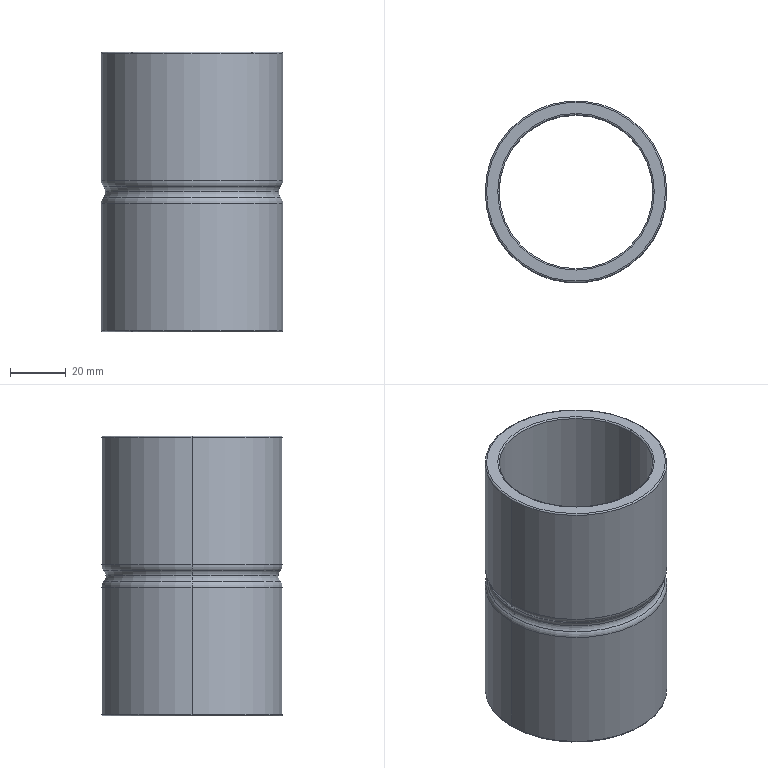Component | SolidWorks | KLHFH007_18LocatingPinSeatBrassSleeve-1 | 1 solid | 24 faces | box 65 x 65 x 100 mm | volume 93014 mm3 | torus 16 | cylinder 6 | plane 2 | commonest cylinder face diameters 65 x4 55 x2 | material Brass
build123d program:
from build123d import *

# Parameters (mm, degrees)
SKETCH1_R           = 32.5
SKETCH1_R_2         = 27.5
BOSS_EXTRUDE1_DEPTH = 50
SKETCH2_R           = 3
FILLET1_R           = 0.5
FILLET2_R           = 3


with BuildPart() as part:
    # Sketch1 → Boss-Extrude1 (new, symmetric)
    with BuildSketch(Plane.XY):
        Circle(SKETCH1_R)
        Circle(SKETCH1_R_2, mode=Mode.SUBTRACT)
    extrude(amount=BOSS_EXTRUDE1_DEPTH, both=True)

    # Sketch2 → Cut-Revolve1 (revolve, cut)
    with BuildSketch(Plane(origin=(0, 0, 0), x_dir=(0, 0, -1), z_dir=(1, 0, 0)), mode=Mode.PRIVATE) as cut_revolve1_sk:
        with Locations((0, 34)):
            Circle(SKETCH2_R)
    revolve(cut_revolve1_sk.sketch.rotate(Axis((0, 0, 0), (0, 0, 1)), 90), axis=Axis((0, 0, 0), (0, 0, 1)), mode=Mode.SUBTRACT)

    # Fillet1
    fillet1_edges = [part.edges().sort_by_distance(p)[0] for p in [
        (-32.5, 0, -50),
        (-32.5, 0, 50),
        (-27.5, 0, -50),
        (-27.5, 0, 50),
    ]]
    fillet(fillet1_edges, radius=FILLET1_R)

    # Fillet2
    fillet2_edges = [part.edges().sort_by_distance(p)[0] for p in [
        (0, 32.5, 2.598),
        (0, 32.5, -2.598),
    ]]
    fillet(fillet2_edges, radius=FILLET2_R)


solid = part.part

# Placed as in the assembly
solid = solid.moved(Location((91, 157.617, -294.5), (0, 0, 0)))
STEP:
#1=CARTESIAN_POINT('',(2.333,6.205,-11.673));
#2=VERTEX_POINT('',#1);
#3=CARTESIAN_POINT('',(2.362,6.205,-11.594));
#4=VERTEX_POINT('',#3);
#5=CARTESIAN_POINT('',(2.244,6.205,-11.594));
#6=DIRECTION('',(0.,-1.,0.));
#7=DIRECTION('',(0.,0.,-1.));
#8=AXIS2_PLACEMENT_3D('',#5,#6,#7);
#9=CIRCLE('',#8,0.1181);
#10=EDGE_CURVE('',#2,#4,#9,.T.);
#11=ORIENTED_EDGE('',*,*,#10,.T.);
#12=CARTESIAN_POINT('',(4.803,6.205,-11.594));
#13=VERTEX_POINT('',#12);
#14=CARTESIAN_POINT('',(3.583,6.205,-11.594));
#15=DIRECTION('',(0.,0.,-1.));
#16=DIRECTION('',(-1.,0.,0.));
#17=AXIS2_PLACEMENT_3D('',#14,#15,#16);
#18=CIRCLE('',#17,1.22);
#19=EDGE_CURVE('',#4,#13,#18,.T.);
#20=ORIENTED_EDGE('',*,*,#19,.T.);
#21=CARTESIAN_POINT('',(4.833,6.205,-11.673));
#22=VERTEX_POINT('',#21);
#23=CARTESIAN_POINT('',(4.921,6.205,-11.594));
#24=DIRECTION('',(-0.,1.,0.));
#25=DIRECTION('',(-1.,0.,0.));
#26=AXIS2_PLACEMENT_3D('',#23,#24,#25);
#27=CIRCLE('',#26,0.1181);
#28=EDGE_CURVE('',#22,#13,#27,.T.);
#29=ORIENTED_EDGE('',*,*,#28,.F.);
#30=CARTESIAN_POINT('',(3.583,6.205,-11.673));
#31=DIRECTION('',(0.,0.,1.));
#32=DIRECTION('',(1.,0.,0.));
#33=AXIS2_PLACEMENT_3D('',#30,#31,#32);
#34=CIRCLE('',#33,1.25);
#35=EDGE_CURVE('',#22,#2,#34,.T.);
#36=ORIENTED_EDGE('',*,*,#35,.T.);
#37=EDGE_LOOP('',(#11,#20,#29,#36));
#38=FACE_OUTER_BOUND('',#37,.T.);
#39=CARTESIAN_POINT('',(3.583,6.205,-11.594));
#40=DIRECTION('',(0.,0.,-1.));
#41=DIRECTION('',(-1.,0.,0.));
#42=AXIS2_PLACEMENT_3D('',#39,#40,#41);
#43=TOROIDAL_SURFACE('',#42,1.339,0.1181);
#44=ADVANCED_FACE('',(#38),#43,.F.);
#45=ORIENTED_EDGE('',*,*,#28,.T.);
#46=CARTESIAN_POINT('',(3.583,6.205,-11.594));
#47=DIRECTION('',(0.,0.,-1.));
#48=DIRECTION('',(-1.,0.,0.));
#49=AXIS2_PLACEMENT_3D('',#46,#47,#48);
#50=CIRCLE('',#49,1.22);
#51=EDGE_CURVE('',#13,#4,#50,.T.);
#52=ORIENTED_EDGE('',*,*,#51,.T.);
#53=ORIENTED_EDGE('',*,*,#10,.F.);
#54=CARTESIAN_POINT('',(3.583,6.205,-11.673));
#55=DIRECTION('',(0.,0.,1.));
#56=DIRECTION('',(1.,0.,0.));
#57=AXIS2_PLACEMENT_3D('',#54,#55,#56);
#58=CIRCLE('',#57,1.25);
#59=EDGE_CURVE('',#2,#22,#58,.T.);
#60=ORIENTED_EDGE('',*,*,#59,.T.);
#61=EDGE_LOOP('',(#45,#52,#53,#60));
#62=FACE_OUTER_BOUND('',#61,.T.);
#63=CARTESIAN_POINT('',(3.583,6.205,-11.594));
#64=DIRECTION('',(0.,0.,-1.));
#65=DIRECTION('',(-1.,0.,0.));
#66=AXIS2_PLACEMENT_3D('',#63,#64,#65);
#67=TOROIDAL_SURFACE('',#66,1.339,0.1181);
#68=ADVANCED_FACE('',(#62),#67,.F.);
#69=CARTESIAN_POINT('',(2.303,6.205,-11.751));
#70=VERTEX_POINT('',#69);
#71=CARTESIAN_POINT('',(4.862,6.205,-11.751));
#72=VERTEX_POINT('',#71);
#73=CARTESIAN_POINT('',(3.583,6.205,-11.751));
#74=DIRECTION('',(0.,0.,-1.));
#75=DIRECTION('',(1.,0.,0.));
#76=AXIS2_PLACEMENT_3D('',#73,#74,#75);
#77=CIRCLE('',#76,1.28);
#78=EDGE_CURVE('',#70,#72,#77,.T.);
#79=ORIENTED_EDGE('',*,*,#78,.F.);
#80=CARTESIAN_POINT('',(2.421,6.205,-11.751));
#81=DIRECTION('',(0.,1.,0.));
#82=DIRECTION('',(-1.,0.,0.));
#83=AXIS2_PLACEMENT_3D('',#80,#81,#82);
#84=CIRCLE('',#83,0.1181);
#85=EDGE_CURVE('',#70,#2,#84,.T.);
#86=ORIENTED_EDGE('',*,*,#85,.T.);
#87=ORIENTED_EDGE('',*,*,#35,.F.);
#88=CARTESIAN_POINT('',(4.744,6.205,-11.751));
#89=DIRECTION('',(0.,-1.,0.));
#90=DIRECTION('',(0.,0.,-1.));
#91=AXIS2_PLACEMENT_3D('',#88,#89,#90);
#92=CIRCLE('',#91,0.1181);
#93=EDGE_CURVE('',#72,#22,#92,.T.);
#94=ORIENTED_EDGE('',*,*,#93,.F.);
#95=EDGE_LOOP('',(#79,#86,#87,#94));
#96=FACE_OUTER_BOUND('',#95,.T.);
#97=CARTESIAN_POINT('',(3.583,6.205,-11.751));
#98=DIRECTION('',(0.,0.,1.));
#99=DIRECTION('',(1.,0.,0.));
#100=AXIS2_PLACEMENT_3D('',#97,#98,#99);
#101=TOROIDAL_SURFACE('',#100,1.161,0.1181);
#102=ADVANCED_FACE('',(#96),#101,.T.);
#103=CARTESIAN_POINT('',(4.862,6.205,-11.438));
#104=VERTEX_POINT('',#103);
#105=CARTESIAN_POINT('',(2.303,6.205,-11.438));
#106=VERTEX_POINT('',#105);
#107=CARTESIAN_POINT('',(3.583,6.205,-11.438));
#108=DIRECTION('',(0.,0.,1.));
#109=DIRECTION('',(-1.,0.,0.));
#110=AXIS2_PLACEMENT_3D('',#107,#108,#109);
#111=CIRCLE('',#110,1.28);
#112=EDGE_CURVE('',#104,#106,#111,.T.);
#113=ORIENTED_EDGE('',*,*,#112,.F.);
#114=CARTESIAN_POINT('',(4.833,6.205,-11.516));
#115=VERTEX_POINT('',#114);
#116=CARTESIAN_POINT('',(4.744,6.205,-11.438));
#117=DIRECTION('',(-0.,1.,0.));
#118=DIRECTION('',(-1.,0.,0.));
#119=AXIS2_PLACEMENT_3D('',#116,#117,#118);
#120=CIRCLE('',#119,0.1181);
#121=EDGE_CURVE('',#104,#115,#120,.T.);
#122=ORIENTED_EDGE('',*,*,#121,.T.);
#123=CARTESIAN_POINT('',(2.333,6.205,-11.516));
#124=VERTEX_POINT('',#123);
#125=CARTESIAN_POINT('',(3.583,6.205,-11.516));
#126=DIRECTION('',(0.,0.,-1.));
#127=DIRECTION('',(-1.,0.,0.));
#128=AXIS2_PLACEMENT_3D('',#125,#126,#127);
#129=CIRCLE('',#128,1.25);
#130=EDGE_CURVE('',#124,#115,#129,.T.);
#131=ORIENTED_EDGE('',*,*,#130,.F.);
#132=CARTESIAN_POINT('',(2.421,6.205,-11.438));
#133=DIRECTION('',(0.,-1.,0.));
#134=DIRECTION('',(0.,0.,-1.));
#135=AXIS2_PLACEMENT_3D('',#132,#133,#134);
#136=CIRCLE('',#135,0.1181);
#137=EDGE_CURVE('',#106,#124,#136,.T.);
#138=ORIENTED_EDGE('',*,*,#137,.F.);
#139=EDGE_LOOP('',(#113,#122,#131,#138));
#140=FACE_OUTER_BOUND('',#139,.T.);
#141=CARTESIAN_POINT('',(3.583,6.205,-11.438));
#142=DIRECTION('',(0.,0.,-1.));
#143=DIRECTION('',(-1.,0.,0.));
#144=AXIS2_PLACEMENT_3D('',#141,#142,#143);
#145=TOROIDAL_SURFACE('',#144,1.161,0.1181);
#146=ADVANCED_FACE('',(#140),#145,.T.);
#147=CARTESIAN_POINT('',(2.303,6.205,-9.646));
#148=VERTEX_POINT('',#147);
#149=CARTESIAN_POINT('',(4.862,6.205,-9.646));
#150=VERTEX_POINT('',#149);
#151=CARTESIAN_POINT('',(3.583,6.205,-9.646));
#152=DIRECTION('',(0.,0.,-1.));
#153=DIRECTION('',(1.,0.,0.));
#154=AXIS2_PLACEMENT_3D('',#151,#152,#153);
#155=CIRCLE('',#154,1.28);
#156=EDGE_CURVE('',#148,#150,#155,.T.);
#157=ORIENTED_EDGE('',*,*,#156,.F.);
#158=CARTESIAN_POINT('',(2.323,6.205,-9.626));
#159=VERTEX_POINT('',#158);
#160=CARTESIAN_POINT('',(2.323,6.205,-9.646));
#161=DIRECTION('',(0.,1.,0.));
#162=DIRECTION('',(-1.,0.,0.));
#163=AXIS2_PLACEMENT_3D('',#160,#161,#162);
#164=CIRCLE('',#163,0.01969);
#165=EDGE_CURVE('',#148,#159,#164,.T.);
#166=ORIENTED_EDGE('',*,*,#165,.T.);
#167=CARTESIAN_POINT('',(4.843,6.205,-9.626));
#168=VERTEX_POINT('',#167);
#169=CARTESIAN_POINT('',(3.583,6.205,-9.626));
#170=DIRECTION('',(0.,0.,1.));
#171=DIRECTION('',(1.,0.,0.));
#172=AXIS2_PLACEMENT_3D('',#169,#170,#171);
#173=CIRCLE('',#172,1.26);
#174=EDGE_CURVE('',#168,#159,#173,.T.);
#175=ORIENTED_EDGE('',*,*,#174,.F.);
#176=CARTESIAN_POINT('',(4.843,6.205,-9.646));
#177=DIRECTION('',(0.,-1.,0.));
#178=DIRECTION('',(0.,0.,-1.));
#179=AXIS2_PLACEMENT_3D('',#176,#177,#178);
#180=CIRCLE('',#179,0.01969);
#181=EDGE_CURVE('',#150,#168,#180,.T.);
#182=ORIENTED_EDGE('',*,*,#181,.F.);
#183=EDGE_LOOP('',(#157,#166,#175,#182));
#184=FACE_OUTER_BOUND('',#183,.T.);
#185=CARTESIAN_POINT('',(3.583,6.205,-9.646));
#186=DIRECTION('',(0.,0.,1.));
#187=DIRECTION('',(1.,0.,0.));
#188=AXIS2_PLACEMENT_3D('',#185,#186,#187);
#189=TOROIDAL_SURFACE('',#188,1.26,0.01969);
#190=ADVANCED_FACE('',(#184),#189,.T.);
#191=CARTESIAN_POINT('',(2.48,6.205,-9.626));
#192=VERTEX_POINT('',#191);
#193=CARTESIAN_POINT('',(4.685,6.205,-9.626));
#194=VERTEX_POINT('',#193);
#195=CARTESIAN_POINT('',(3.583,6.205,-9.626));
#196=DIRECTION('',(0.,0.,-1.));
#197=DIRECTION('',(1.,0.,0.));
#198=AXIS2_PLACEMENT_3D('',#195,#196,#197);
#199=CIRCLE('',#198,1.102);
#200=EDGE_CURVE('',#192,#194,#199,.T.);
#201=ORIENTED_EDGE('',*,*,#200,.F.);
#202=CARTESIAN_POINT('',(2.5,6.205,-9.646));
#203=VERTEX_POINT('',#202);
#204=CARTESIAN_POINT('',(2.48,6.205,-9.646));
#205=DIRECTION('',(0.,1.,0.));
#206=DIRECTION('',(-1.,0.,0.));
#207=AXIS2_PLACEMENT_3D('',#204,#205,#206);
#208=CIRCLE('',#207,0.01969);
#209=EDGE_CURVE('',#192,#203,#208,.T.);
#210=ORIENTED_EDGE('',*,*,#209,.T.);
#211=CARTESIAN_POINT('',(4.665,6.205,-9.646));
#212=VERTEX_POINT('',#211);
#213=CARTESIAN_POINT('',(3.583,6.205,-9.646));
#214=DIRECTION('',(0.,0.,1.));
#215=DIRECTION('',(1.,0.,0.));
#216=AXIS2_PLACEMENT_3D('',#213,#214,#215);
#217=CIRCLE('',#216,1.083);
#218=EDGE_CURVE('',#212,#203,#217,.T.);
#219=ORIENTED_EDGE('',*,*,#218,.F.);
#220=CARTESIAN_POINT('',(4.685,6.205,-9.646));
#221=DIRECTION('',(0.,-1.,0.));
#222=DIRECTION('',(0.,0.,-1.));
#223=AXIS2_PLACEMENT_3D('',#220,#221,#222);
#224=CIRCLE('',#223,0.01969);
#225=EDGE_CURVE('',#194,#212,#224,.T.);
#226=ORIENTED_EDGE('',*,*,#225,.F.);
#227=EDGE_LOOP('',(#201,#210,#219,#226));
#228=FACE_OUTER_BOUND('',#227,.T.);
#229=CARTESIAN_POINT('',(3.583,6.205,-9.646));
#230=DIRECTION('',(0.,0.,1.));
#231=DIRECTION('',(1.,0.,0.));
#232=AXIS2_PLACEMENT_3D('',#229,#230,#231);
#233=TOROIDAL_SURFACE('',#232,1.102,0.01969);
#234=ADVANCED_FACE('',(#228),#233,.T.);
#235=CARTESIAN_POINT('',(2.323,6.205,-13.563));
#236=VERTEX_POINT('',#235);
#237=CARTESIAN_POINT('',(4.843,6.205,-13.563));
#238=VERTEX_POINT('',#237);
#239=CARTESIAN_POINT('',(3.583,6.205,-13.563));
#240=DIRECTION('',(0.,0.,-1.));
#241=DIRECTION('',(1.,0.,0.));
#242=AXIS2_PLACEMENT_3D('',#239,#240,#241);
#243=CIRCLE('',#242,1.26);
#244=EDGE_CURVE('',#236,#238,#243,.T.);
#245=ORIENTED_EDGE('',*,*,#244,.F.);
#246=CARTESIAN_POINT('',(2.303,6.205,-13.543));
#247=VERTEX_POINT('',#246);
#248=CARTESIAN_POINT('',(2.323,6.205,-13.543));
#249=DIRECTION('',(0.,1.,0.));
#250=DIRECTION('',(-1.,0.,0.));
#251=AXIS2_PLACEMENT_3D('',#248,#249,#250);
#252=CIRCLE('',#251,0.01969);
#253=EDGE_CURVE('',#236,#247,#252,.T.);
#254=ORIENTED_EDGE('',*,*,#253,.T.);
#255=CARTESIAN_POINT('',(4.862,6.205,-13.543));
#256=VERTEX_POINT('',#255);
#257=CARTESIAN_POINT('',(3.583,6.205,-13.543));
#258=DIRECTION('',(0.,0.,1.));
#259=DIRECTION('',(1.,0.,0.));
#260=AXIS2_PLACEMENT_3D('',#257,#258,#259);
#261=CIRCLE('',#260,1.28);
#262=EDGE_CURVE('',#256,#247,#261,.T.);
#263=ORIENTED_EDGE('',*,*,#262,.F.);
#264=CARTESIAN_POINT('',(4.843,6.205,-13.543));
#265=DIRECTION('',(0.,-1.,0.));
#266=DIRECTION('',(0.,0.,-1.));
#267=AXIS2_PLACEMENT_3D('',#264,#265,#266);
#268=CIRCLE('',#267,0.01969);
#269=EDGE_CURVE('',#238,#256,#268,.T.);
#270=ORIENTED_EDGE('',*,*,#269,.F.);
#271=EDGE_LOOP('',(#245,#254,#263,#270));
#272=FACE_OUTER_BOUND('',#271,.T.);
#273=CARTESIAN_POINT('',(3.583,6.205,-13.543));
#274=DIRECTION('',(0.,0.,1.));
#275=DIRECTION('',(1.,0.,0.));
#276=AXIS2_PLACEMENT_3D('',#273,#274,#275);
#277=TOROIDAL_SURFACE('',#276,1.26,0.01969);
#278=ADVANCED_FACE('',(#272),#277,.T.);
#279=CARTESIAN_POINT('',(2.5,6.205,-13.543));
#280=VERTEX_POINT('',#279);
#281=CARTESIAN_POINT('',(4.665,6.205,-13.543));
#282=VERTEX_POINT('',#281);
#283=CARTESIAN_POINT('',(3.583,6.205,-13.543));
#284=DIRECTION('',(0.,0.,-1.));
#285=DIRECTION('',(1.,0.,0.));
#286=AXIS2_PLACEMENT_3D('',#283,#284,#285);
#287=CIRCLE('',#286,1.083);
#288=EDGE_CURVE('',#280,#282,#287,.T.);
#289=ORIENTED_EDGE('',*,*,#288,.F.);
#290=CARTESIAN_POINT('',(2.48,6.205,-13.563));
#291=VERTEX_POINT('',#290);
#292=CARTESIAN_POINT('',(2.48,6.205,-13.543));
#293=DIRECTION('',(0.,1.,0.));
#294=DIRECTION('',(-1.,0.,0.));
#295=AXIS2_PLACEMENT_3D('',#292,#293,#294);
#296=CIRCLE('',#295,0.01969);
#297=EDGE_CURVE('',#280,#291,#296,.T.);
#298=ORIENTED_EDGE('',*,*,#297,.T.);
#299=CARTESIAN_POINT('',(4.685,6.205,-13.563));
#300=VERTEX_POINT('',#299);
#301=CARTESIAN_POINT('',(3.583,6.205,-13.563));
#302=DIRECTION('',(0.,0.,1.));
#303=DIRECTION('',(1.,0.,0.));
#304=AXIS2_PLACEMENT_3D('',#301,#302,#303);
#305=CIRCLE('',#304,1.102);
#306=EDGE_CURVE('',#300,#291,#305,.T.);
#307=ORIENTED_EDGE('',*,*,#306,.F.);
#308=CARTESIAN_POINT('',(4.685,6.205,-13.543));
#309=DIRECTION('',(0.,-1.,0.));
#310=DIRECTION('',(0.,0.,-1.));
#311=AXIS2_PLACEMENT_3D('',#308,#309,#310);
#312=CIRCLE('',#311,0.01969);
#313=EDGE_CURVE('',#282,#300,#312,.T.);
#314=ORIENTED_EDGE('',*,*,#313,.F.);
#315=EDGE_LOOP('',(#289,#298,#307,#314));
#316=FACE_OUTER_BOUND('',#315,.T.);
#317=CARTESIAN_POINT('',(3.583,6.205,-13.543));
#318=DIRECTION('',(0.,0.,1.));
#319=DIRECTION('',(1.,0.,0.));
#320=AXIS2_PLACEMENT_3D('',#317,#318,#319);
#321=TOROIDAL_SURFACE('',#320,1.102,0.01969);
#322=ADVANCED_FACE('',(#316),#321,.T.);
#323=ORIENTED_EDGE('',*,*,#51,.F.);
#324=CARTESIAN_POINT('',(4.921,6.205,-11.594));
#325=DIRECTION('',(-0.,1.,0.));
#326=DIRECTION('',(-1.,0.,0.));
#327=AXIS2_PLACEMENT_3D('',#324,#325,#326);
#328=CIRCLE('',#327,0.1181);
#329=EDGE_CURVE('',#13,#115,#328,.T.);
#330=ORIENTED_EDGE('',*,*,#329,.T.);
#331=CARTESIAN_POINT('',(3.583,6.205,-11.516));
#332=DIRECTION('',(0.,0.,-1.));
#333=DIRECTION('',(-1.,0.,0.));
#334=AXIS2_PLACEMENT_3D('',#331,#332,#333);
#335=CIRCLE('',#334,1.25);
#336=EDGE_CURVE('',#115,#124,#335,.T.);
#337=ORIENTED_EDGE('',*,*,#336,.T.);
#338=CARTESIAN_POINT('',(2.244,6.205,-11.594));
#339=DIRECTION('',(0.,-1.,0.));
#340=DIRECTION('',(0.,0.,-1.));
#341=AXIS2_PLACEMENT_3D('',#338,#339,#340);
#342=CIRCLE('',#341,0.1181);
#343=EDGE_CURVE('',#4,#124,#342,.T.);
#344=ORIENTED_EDGE('',*,*,#343,.F.);
#345=EDGE_LOOP('',(#323,#330,#337,#344));
#346=FACE_OUTER_BOUND('',#345,.T.);
#347=CARTESIAN_POINT('',(3.583,6.205,-11.594));
#348=DIRECTION('',(0.,0.,-1.));
#349=DIRECTION('',(-1.,0.,0.));
#350=AXIS2_PLACEMENT_3D('',#347,#348,#349);
#351=TOROIDAL_SURFACE('',#350,1.339,0.1181);
#352=ADVANCED_FACE('',(#346),#351,.F.);
#353=CARTESIAN_POINT('',(3.583,6.205,-9.646));
#354=DIRECTION('',(0.,0.,1.));
#355=DIRECTION('',(1.,0.,0.));
#356=AXIS2_PLACEMENT_3D('',#353,#354,#355);
#357=CIRCLE('',#356,1.083);
#358=EDGE_CURVE('',#203,#212,#357,.T.);
#359=ORIENTED_EDGE('',*,*,#358,.T.);
#360=CARTESIAN_POINT('',(4.665,6.205,-9.626));
#361=DIRECTION('',(0.,0.,-1.));
#362=VECTOR('',#361,39.37);
#363=LINE('',#360,#362);
#364=EDGE_CURVE('',#212,#282,#363,.T.);
#365=ORIENTED_EDGE('',*,*,#364,.T.);
#366=CARTESIAN_POINT('',(3.583,6.205,-13.543));
#367=DIRECTION('',(0.,0.,-1.));
#368=DIRECTION('',(1.,0.,0.));
#369=AXIS2_PLACEMENT_3D('',#366,#367,#368);
#370=CIRCLE('',#369,1.083);
#371=EDGE_CURVE('',#282,#280,#370,.T.);
#372=ORIENTED_EDGE('',*,*,#371,.T.);
#373=CARTESIAN_POINT('',(2.5,6.205,-9.626));
#374=DIRECTION('',(0.,0.,-1.));
#375=VECTOR('',#374,39.37);
#376=LINE('',#373,#375);
#377=EDGE_CURVE('',#203,#280,#376,.T.);
#378=ORIENTED_EDGE('',*,*,#377,.F.);
#379=EDGE_LOOP('',(#359,#365,#372,#378));
#380=FACE_OUTER_BOUND('',#379,.T.);
#381=CARTESIAN_POINT('',(3.583,6.205,-9.626));
#382=DIRECTION('',(0.,0.,-1.));
#383=DIRECTION('',(-1.,0.,0.));
#384=AXIS2_PLACEMENT_3D('',#381,#382,#383);
#385=CYLINDRICAL_SURFACE('',#384,1.083);
#386=ADVANCED_FACE('',(#380),#385,.F.);
#387=ORIENTED_EDGE('',*,*,#156,.T.);
#388=CARTESIAN_POINT('',(4.862,6.205,-9.626));
#389=DIRECTION('',(0.,0.,-1.));
#390=VECTOR('',#389,39.37);
#391=LINE('',#388,#390);
#392=EDGE_CURVE('',#150,#104,#391,.T.);
#393=ORIENTED_EDGE('',*,*,#392,.T.);
#394=ORIENTED_EDGE('',*,*,#112,.T.);
#395=CARTESIAN_POINT('',(2.303,6.205,-9.626));
#396=DIRECTION('',(0.,0.,-1.));
#397=VECTOR('',#396,39.37);
#398=LINE('',#395,#397);
#399=EDGE_CURVE('',#148,#106,#398,.T.);
#400=ORIENTED_EDGE('',*,*,#399,.F.);
#401=EDGE_LOOP('',(#387,#393,#394,#400));
#402=FACE_OUTER_BOUND('',#401,.T.);
#403=CARTESIAN_POINT('',(3.583,6.205,-9.626));
#404=DIRECTION('',(0.,0.,-1.));
#405=DIRECTION('',(-1.,0.,0.));
#406=AXIS2_PLACEMENT_3D('',#403,#404,#405);
#407=CYLINDRICAL_SURFACE('',#406,1.28);
#408=ADVANCED_FACE('',(#402),#407,.T.);
#409=ORIENTED_EDGE('',*,*,#78,.T.);
#410=CARTESIAN_POINT('',(4.862,6.205,-9.626));
#411=DIRECTION('',(0.,0.,-1.));
#412=VECTOR('',#411,39.37);
#413=LINE('',#410,#412);
#414=EDGE_CURVE('',#72,#256,#413,.T.);
#415=ORIENTED_EDGE('',*,*,#414,.T.);
#416=ORIENTED_EDGE('',*,*,#262,.T.);
#417=CARTESIAN_POINT('',(2.303,6.205,-9.626));
#418=DIRECTION('',(0.,0.,-1.));
#419=VECTOR('',#418,39.37);
#420=LINE('',#417,#419);
#421=EDGE_CURVE('',#70,#247,#420,.T.);
#422=ORIENTED_EDGE('',*,*,#421,.F.);
#423=EDGE_LOOP('',(#409,#415,#416,#422));
#424=FACE_OUTER_BOUND('',#423,.T.);
#425=CARTESIAN_POINT('',(3.583,6.205,-9.626));
#426=DIRECTION('',(0.,0.,-1.));
#427=DIRECTION('',(-1.,0.,0.));
#428=AXIS2_PLACEMENT_3D('',#425,#426,#427);
#429=CYLINDRICAL_SURFACE('',#428,1.28);
#430=ADVANCED_FACE('',(#424),#429,.T.);
#431=ORIENTED_EDGE('',*,*,#414,.F.);
#432=CARTESIAN_POINT('',(3.583,6.205,-11.751));
#433=DIRECTION('',(0.,0.,-1.));
#434=DIRECTION('',(1.,0.,0.));
#435=AXIS2_PLACEMENT_3D('',#432,#433,#434);
#436=CIRCLE('',#435,1.28);
#437=EDGE_CURVE('',#72,#70,#436,.T.);
#438=ORIENTED_EDGE('',*,*,#437,.T.);
#439=ORIENTED_EDGE('',*,*,#421,.T.);
#440=CARTESIAN_POINT('',(3.583,6.205,-13.543));
#441=DIRECTION('',(0.,0.,1.));
#442=DIRECTION('',(1.,0.,0.));
#443=AXIS2_PLACEMENT_3D('',#440,#441,#442);
#444=CIRCLE('',#443,1.28);
#445=EDGE_CURVE('',#247,#256,#444,.T.);
#446=ORIENTED_EDGE('',*,*,#445,.T.);
#447=EDGE_LOOP('',(#431,#438,#439,#446));
#448=FACE_OUTER_BOUND('',#447,.T.);
#449=CARTESIAN_POINT('',(3.583,6.205,-9.626));
#450=DIRECTION('',(0.,0.,-1.));
#451=DIRECTION('',(-1.,0.,0.));
#452=AXIS2_PLACEMENT_3D('',#449,#450,#451);
#453=CYLINDRICAL_SURFACE('',#452,1.28);
#454=ADVANCED_FACE('',(#448),#453,.T.);
#455=CARTESIAN_POINT('',(3.583,6.205,-9.626));
#456=DIRECTION('',(0.,0.,-1.));
#457=DIRECTION('',(1.,0.,0.));
#458=AXIS2_PLACEMENT_3D('',#455,#456,#457);
#459=CIRCLE('',#458,1.102);
#460=EDGE_CURVE('',#194,#192,#459,.T.);
#461=ORIENTED_EDGE('',*,*,#460,.T.);
#462=ORIENTED_EDGE('',*,*,#200,.T.);
#463=EDGE_LOOP('',(#461,#462));
#464=FACE_BOUND('',#463,.T.);
#465=ORIENTED_EDGE('',*,*,#174,.T.);
#466=CARTESIAN_POINT('',(3.583,6.205,-9.626));
#467=DIRECTION('',(0.,0.,1.));
#468=DIRECTION('',(1.,0.,0.));
#469=AXIS2_PLACEMENT_3D('',#466,#467,#468);
#470=CIRCLE('',#469,1.26);
#471=EDGE_CURVE('',#159,#168,#470,.T.);
#472=ORIENTED_EDGE('',*,*,#471,.T.);
#473=EDGE_LOOP('',(#465,#472));
#474=FACE_OUTER_BOUND('',#473,.T.);
#475=CARTESIAN_POINT('',(3.583,6.205,-9.626));
#476=DIRECTION('',(0.,0.,1.));
#477=DIRECTION('',(1.,0.,0.));
#478=AXIS2_PLACEMENT_3D('',#475,#476,#477);
#479=PLANE('',#478);
#480=ADVANCED_FACE('',(#464,#474),#479,.T.);
#481=ORIENTED_EDGE('',*,*,#306,.T.);
#482=CARTESIAN_POINT('',(3.583,6.205,-13.563));
#483=DIRECTION('',(0.,0.,1.));
#484=DIRECTION('',(1.,0.,0.));
#485=AXIS2_PLACEMENT_3D('',#482,#483,#484);
#486=CIRCLE('',#485,1.102);
#487=EDGE_CURVE('',#291,#300,#486,.T.);
#488=ORIENTED_EDGE('',*,*,#487,.T.);
#489=EDGE_LOOP('',(#481,#488));
#490=FACE_BOUND('',#489,.T.);
#491=CARTESIAN_POINT('',(3.583,6.205,-13.563));
#492=DIRECTION('',(0.,0.,-1.));
#493=DIRECTION('',(1.,0.,0.));
#494=AXIS2_PLACEMENT_3D('',#491,#492,#493);
#495=CIRCLE('',#494,1.26);
#496=EDGE_CURVE('',#238,#236,#495,.T.);
#497=ORIENTED_EDGE('',*,*,#496,.T.);
#498=ORIENTED_EDGE('',*,*,#244,.T.);
#499=EDGE_LOOP('',(#497,#498));
#500=FACE_OUTER_BOUND('',#499,.T.);
#501=CARTESIAN_POINT('',(3.583,6.205,-13.563));
#502=DIRECTION('',(0.,0.,1.));
#503=DIRECTION('',(1.,0.,0.));
#504=AXIS2_PLACEMENT_3D('',#501,#502,#503);
#505=PLANE('',#504);
#506=ADVANCED_FACE('',(#490,#500),#505,.F.);
#507=ORIENTED_EDGE('',*,*,#392,.F.);
#508=CARTESIAN_POINT('',(3.583,6.205,-9.646));
#509=DIRECTION('',(0.,0.,-1.));
#510=DIRECTION('',(1.,0.,0.));
#511=AXIS2_PLACEMENT_3D('',#508,#509,#510);
#512=CIRCLE('',#511,1.28);
#513=EDGE_CURVE('',#150,#148,#512,.T.);
#514=ORIENTED_EDGE('',*,*,#513,.T.);
#515=ORIENTED_EDGE('',*,*,#399,.T.);
#516=CARTESIAN_POINT('',(3.583,6.205,-11.438));
#517=DIRECTION('',(0.,0.,1.));
#518=DIRECTION('',(-1.,0.,0.));
#519=AXIS2_PLACEMENT_3D('',#516,#517,#518);
#520=CIRCLE('',#519,1.28);
#521=EDGE_CURVE('',#106,#104,#520,.T.);
#522=ORIENTED_EDGE('',*,*,#521,.T.);
#523=EDGE_LOOP('',(#507,#514,#515,#522));
#524=FACE_OUTER_BOUND('',#523,.T.);
#525=CARTESIAN_POINT('',(3.583,6.205,-9.626));
#526=DIRECTION('',(0.,0.,-1.));
#527=DIRECTION('',(-1.,0.,0.));
#528=AXIS2_PLACEMENT_3D('',#525,#526,#527);
#529=CYLINDRICAL_SURFACE('',#528,1.28);
#530=ADVANCED_FACE('',(#524),#529,.T.);
#531=ORIENTED_EDGE('',*,*,#364,.F.);
#532=ORIENTED_EDGE('',*,*,#218,.T.);
#533=ORIENTED_EDGE('',*,*,#377,.T.);
#534=ORIENTED_EDGE('',*,*,#288,.T.);
#535=EDGE_LOOP('',(#531,#532,#533,#534));
#536=FACE_OUTER_BOUND('',#535,.T.);
#537=CARTESIAN_POINT('',(3.583,6.205,-9.626));
#538=DIRECTION('',(0.,0.,-1.));
#539=DIRECTION('',(-1.,0.,0.));
#540=AXIS2_PLACEMENT_3D('',#537,#538,#539);
#541=CYLINDRICAL_SURFACE('',#540,1.083);
#542=ADVANCED_FACE('',(#536),#541,.F.);
#543=ORIENTED_EDGE('',*,*,#19,.F.);
#544=ORIENTED_EDGE('',*,*,#343,.T.);
#545=ORIENTED_EDGE('',*,*,#130,.T.);
#546=ORIENTED_EDGE('',*,*,#329,.F.);
#547=EDGE_LOOP('',(#543,#544,#545,#546));
#548=FACE_OUTER_BOUND('',#547,.T.);
#549=CARTESIAN_POINT('',(3.583,6.205,-11.594));
#550=DIRECTION('',(0.,0.,-1.));
#551=DIRECTION('',(-1.,0.,0.));
#552=AXIS2_PLACEMENT_3D('',#549,#550,#551);
#553=TOROIDAL_SURFACE('',#552,1.339,0.1181);
#554=ADVANCED_FACE('',(#548),#553,.F.);
#555=ORIENTED_EDGE('',*,*,#297,.F.);
#556=ORIENTED_EDGE('',*,*,#371,.F.);
#557=ORIENTED_EDGE('',*,*,#313,.T.);
#558=ORIENTED_EDGE('',*,*,#487,.F.);
#559=EDGE_LOOP('',(#555,#556,#557,#558));
#560=FACE_OUTER_BOUND('',#559,.T.);
#561=CARTESIAN_POINT('',(3.583,6.205,-13.543));
#562=DIRECTION('',(0.,0.,1.));
#563=DIRECTION('',(1.,0.,0.));
#564=AXIS2_PLACEMENT_3D('',#561,#562,#563);
#565=TOROIDAL_SURFACE('',#564,1.102,0.01969);
#566=ADVANCED_FACE('',(#560),#565,.T.);
#567=ORIENTED_EDGE('',*,*,#253,.F.);
#568=ORIENTED_EDGE('',*,*,#496,.F.);
#569=ORIENTED_EDGE('',*,*,#269,.T.);
#570=ORIENTED_EDGE('',*,*,#445,.F.);
#571=EDGE_LOOP('',(#567,#568,#569,#570));
#572=FACE_OUTER_BOUND('',#571,.T.);
#573=CARTESIAN_POINT('',(3.583,6.205,-13.543));
#574=DIRECTION('',(0.,0.,1.));
#575=DIRECTION('',(1.,0.,0.));
#576=AXIS2_PLACEMENT_3D('',#573,#574,#575);
#577=TOROIDAL_SURFACE('',#576,1.26,0.01969);
#578=ADVANCED_FACE('',(#572),#577,.T.);
#579=ORIENTED_EDGE('',*,*,#209,.F.);
#580=ORIENTED_EDGE('',*,*,#460,.F.);
#581=ORIENTED_EDGE('',*,*,#225,.T.);
#582=ORIENTED_EDGE('',*,*,#358,.F.);
#583=EDGE_LOOP('',(#579,#580,#581,#582));
#584=FACE_OUTER_BOUND('',#583,.T.);
#585=CARTESIAN_POINT('',(3.583,6.205,-9.646));
#586=DIRECTION('',(0.,0.,1.));
#587=DIRECTION('',(1.,0.,0.));
#588=AXIS2_PLACEMENT_3D('',#585,#586,#587);
#589=TOROIDAL_SURFACE('',#588,1.102,0.01969);
#590=ADVANCED_FACE('',(#584),#589,.T.);
#591=ORIENTED_EDGE('',*,*,#165,.F.);
#592=ORIENTED_EDGE('',*,*,#513,.F.);
#593=ORIENTED_EDGE('',*,*,#181,.T.);
#594=ORIENTED_EDGE('',*,*,#471,.F.);
#595=EDGE_LOOP('',(#591,#592,#593,#594));
#596=FACE_OUTER_BOUND('',#595,.T.);
#597=CARTESIAN_POINT('',(3.583,6.205,-9.646));
#598=DIRECTION('',(0.,0.,1.));
#599=DIRECTION('',(1.,0.,0.));
#600=AXIS2_PLACEMENT_3D('',#597,#598,#599);
#601=TOROIDAL_SURFACE('',#600,1.26,0.01969);
#602=ADVANCED_FACE('',(#596),#601,.T.);
#603=ORIENTED_EDGE('',*,*,#121,.F.);
#604=ORIENTED_EDGE('',*,*,#521,.F.);
#605=ORIENTED_EDGE('',*,*,#137,.T.);
#606=ORIENTED_EDGE('',*,*,#336,.F.);
#607=EDGE_LOOP('',(#603,#604,#605,#606));
#608=FACE_OUTER_BOUND('',#607,.T.);
#609=CARTESIAN_POINT('',(3.583,6.205,-11.438));
#610=DIRECTION('',(0.,0.,-1.));
#611=DIRECTION('',(-1.,0.,0.));
#612=AXIS2_PLACEMENT_3D('',#609,#610,#611);
#613=TOROIDAL_SURFACE('',#612,1.161,0.1181);
#614=ADVANCED_FACE('',(#608),#613,.T.);
#615=ORIENTED_EDGE('',*,*,#85,.F.);
#616=ORIENTED_EDGE('',*,*,#437,.F.);
#617=ORIENTED_EDGE('',*,*,#93,.T.);
#618=ORIENTED_EDGE('',*,*,#59,.F.);
#619=EDGE_LOOP('',(#615,#616,#617,#618));
#620=FACE_OUTER_BOUND('',#619,.T.);
#621=CARTESIAN_POINT('',(3.583,6.205,-11.751));
#622=DIRECTION('',(0.,0.,1.));
#623=DIRECTION('',(1.,0.,0.));
#624=AXIS2_PLACEMENT_3D('',#621,#622,#623);
#625=TOROIDAL_SURFACE('',#624,1.161,0.1181);
#626=ADVANCED_FACE('',(#620),#625,.T.);
#627=CLOSED_SHELL('',(#44,#68,#102,#146,#190,#234,#278,#322,#352,#386,#408,#430,#454,#480,#506,#530,#542,#554,#566,#578,#590,#602,#614,#626));
#628=MANIFOLD_SOLID_BREP('',#627);
#629=CARTESIAN_POINT('',(0.,0.,0.));
#630=DIRECTION('',(0.,0.,1.));
#631=DIRECTION('',(1.,0.,0.));
#632=AXIS2_PLACEMENT_3D('',#629,#630,#631);
#633=(LENGTH_UNIT()NAMED_UNIT(*)SI_UNIT($,.METRE.));
#634=LENGTH_MEASURE_WITH_UNIT(LENGTH_MEASURE(0.0254),#633);
#635=DIMENSIONAL_EXPONENTS(1.,0.,0.,0.,0.,0.,0.);
#636=(CONVERSION_BASED_UNIT('',#634)LENGTH_UNIT()NAMED_UNIT(#635));
#637=UNCERTAINTY_MEASURE_WITH_UNIT(LENGTH_MEASURE(0.00001),#636,'','');
#638=(NAMED_UNIT(*)PLANE_ANGLE_UNIT()SI_UNIT($,.RADIAN.));
#639=(NAMED_UNIT(*)SI_UNIT($,.STERADIAN.)SOLID_ANGLE_UNIT());
#640=(GEOMETRIC_REPRESENTATION_CONTEXT(3)GLOBAL_UNCERTAINTY_ASSIGNED_CONTEXT((#637))GLOBAL_UNIT_ASSIGNED_CONTEXT((#636,#638,#639))REPRESENTATION_CONTEXT('',''));
#641=ADVANCED_BREP_SHAPE_REPRESENTATION('',(#628,#632),#640);
#642=COLOUR_RGB('',0.7922,0.8196,0.9333);
#643=FILL_AREA_STYLE_COLOUR('',#642);
#644=FILL_AREA_STYLE('',(#643));
#645=SURFACE_STYLE_FILL_AREA(#644);
#646=SURFACE_SIDE_STYLE('',(#645));
#647=SURFACE_STYLE_USAGE(.BOTH.,#646);
#648=PRESENTATION_STYLE_ASSIGNMENT((#647));
#649=STYLED_ITEM('',(#648),#628);
#650=PRESENTATION_LAYER_ASSIGNMENT('','',(#649));
#651=(LENGTH_UNIT()NAMED_UNIT(*)SI_UNIT($,.METRE.));
#652=LENGTH_MEASURE_WITH_UNIT(LENGTH_MEASURE(0.0254),#651);
#653=DIMENSIONAL_EXPONENTS(1.,0.,0.,0.,0.,0.,0.);
#654=(CONVERSION_BASED_UNIT('',#652)LENGTH_UNIT()NAMED_UNIT(#653));
#655=UNCERTAINTY_MEASURE_WITH_UNIT(LENGTH_MEASURE(0.00001),#654,'','');
#656=(NAMED_UNIT(*)PLANE_ANGLE_UNIT()SI_UNIT($,.RADIAN.));
#657=(NAMED_UNIT(*)SI_UNIT($,.STERADIAN.)SOLID_ANGLE_UNIT());
#658=(GEOMETRIC_REPRESENTATION_CONTEXT(3)GLOBAL_UNCERTAINTY_ASSIGNED_CONTEXT((#655))GLOBAL_UNIT_ASSIGNED_CONTEXT((#654,#656,#657))REPRESENTATION_CONTEXT('',''));
#659=MECHANICAL_DESIGN_GEOMETRIC_PRESENTATION_REPRESENTATION('',(#649),#658);